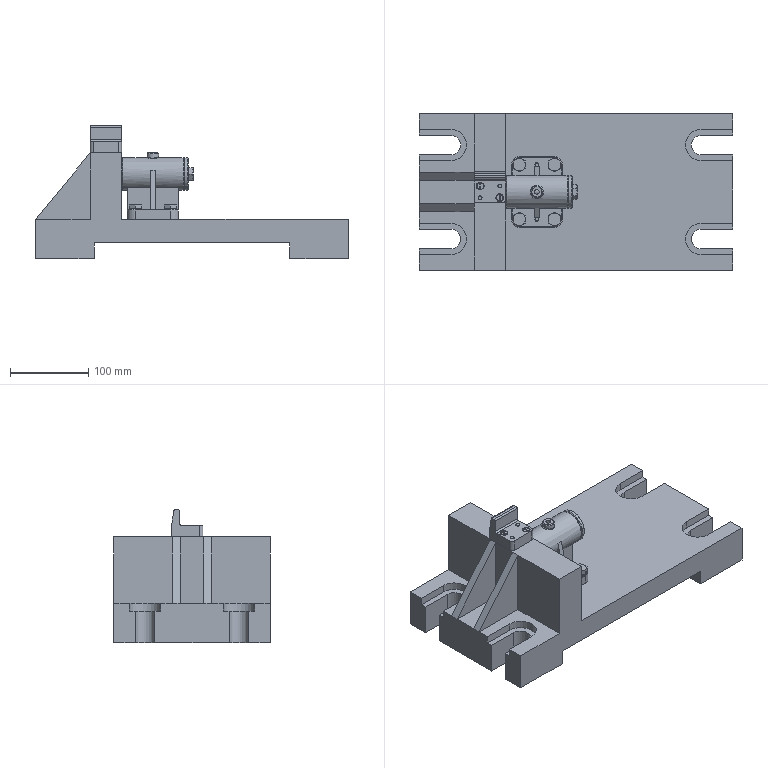Assembly | NX | mm | 20 component files | 20 solids | 442 faces | box 400 x 200 x 170 mm | volume 3663104 mm3 | plane 184 | cylinder 113 | cone 106 | torus 38 | spline 1 | commonest cylinder face diameters 10 x32 5 x22 4 x11 16 x10 2 x8 11 x5 24 x4 40 x4
Bill of materials:
unnamed part 1 | 2 |  | Slotted cylindrical-head screw-like part: short cylindrical head with a single straight slot across the top and a slight taper on the head side, on a long plain cylindrical shank.
unnamed part 2 | 1 |  | Hex-head bolt-like part: hexagonal head with chamfered corners, on a long cylindrical shank with a small step or groove partway along it and a chamfered tip.
unnamed part 3 | 1 |  | L-shaped angle bracket block: rectangular base plate with four through holes and an upright wall along one edge. The wall's outer face is tapered, its top edge is rounded, and there is a fillet where it meets the base.
unnamed part 4 | 4 |  | Hex-head bolt-like part: hexagonal head with chamfered top and a washer face underneath, on a cylindrical shank with a circumferential groove/neck partway along it and a chamfered end.
unnamed part 5 | 1 |  | Flanged bushing/hub: circular flange with four equally spaced through holes, a central through bore, an annular recessed step around the bore on the flange face, and a cylindrical hub on the opposite side.
unnamed part 6 | 2 |  | Solid cylindrical pin with chamfered edges at both ends.
unnamed part 7 | 2 |  | Solid cylindrical pin with chamfered edges at both ends. It looks slightly larger in diameter relative to its length than unnamed part 6.
unnamed part 8 | 5 |  | Plain flat ring (washer/spacer shape) with a rectangular cross-section: concentric circular inner and outer edges and flat faces.
unnamed part 9 | 1 |  | Machined base plate with an integral upright block at one end. The plate has four open-ended U-slots, two at each end, which appear counterbored. The upright has an angled back face, a small protruding cylindrical boss with a hole, and stepped notches on one side. Several small holes are on the plate and upright top, and the underside has a central relief between end pads.
unnamed part 10 | 1 |  | Pillow-block-style housing: horizontal cylindrical barrel with a through bore and four small holes on a bolt circle on its end face. A small cylindrical boss with a hole sits on top. The barrel is carried by tapered webs and a central rib on a rectangular base with rounded corners, four corner holes (counterbored) and two smaller holes. A rectangular relief channel runs under the base.
Mates:
1. fix | fixture_body 1 component
2. align lock | guide_block 1 face | fixture_body 1 face
3. align lock | guide_block 1 face | fixture_body 1 face
4. concentric | guide_block 1 | fixture_body 1
5. concentric | pin_M5x25 1 edge | guide_block 1 edge
6. concentric | pin_M5x25 2 edge | guide_block 1 edge
7. concentric | screw_M5x25 1 edge | guide_block 1 edge
8. concentric | screw_M5x25 2 edge | guide_block 1 edge
9. align lock | bracket 1 face | fixture_body 1 face
10. concentric | bracket 1 edge | fixture_body 1 edge
11. concentric | pin_M5x20 2 edge | bracket 1 edge
12. concentric | pin_M5x20 1 edge | bracket 1 edge
13. concentric | M10_washer 2 edge | bracket 1 edge
14. concentric | M10_washer 4 edge | bracket 1 edge
15. concentric | M10_washer 5 edge | bracket 1 edge
16. concentric | M10_washer 3 edge | bracket 1 edge
17. concentric | bolt_M10x33 4 edge | M10_washer 2 edge
18. concentric | bolt_M10x33 1 edge | M10_washer 4 edge
19. concentric | bolt_M10x33 2 edge | M10_washer 5 edge
20. concentric | bolt_M10x33 3 edge | M10_washer 3 edge
21. align lock | clamp_plate 1 face | bracket 1 face
22. concentric | clamp_plate 1 edge | bracket 1 edge
23. align lock | M10x80 1 face | clamp_plate 1 face
24. concentric | M10x80 1 edge | M10_washer 1 edge